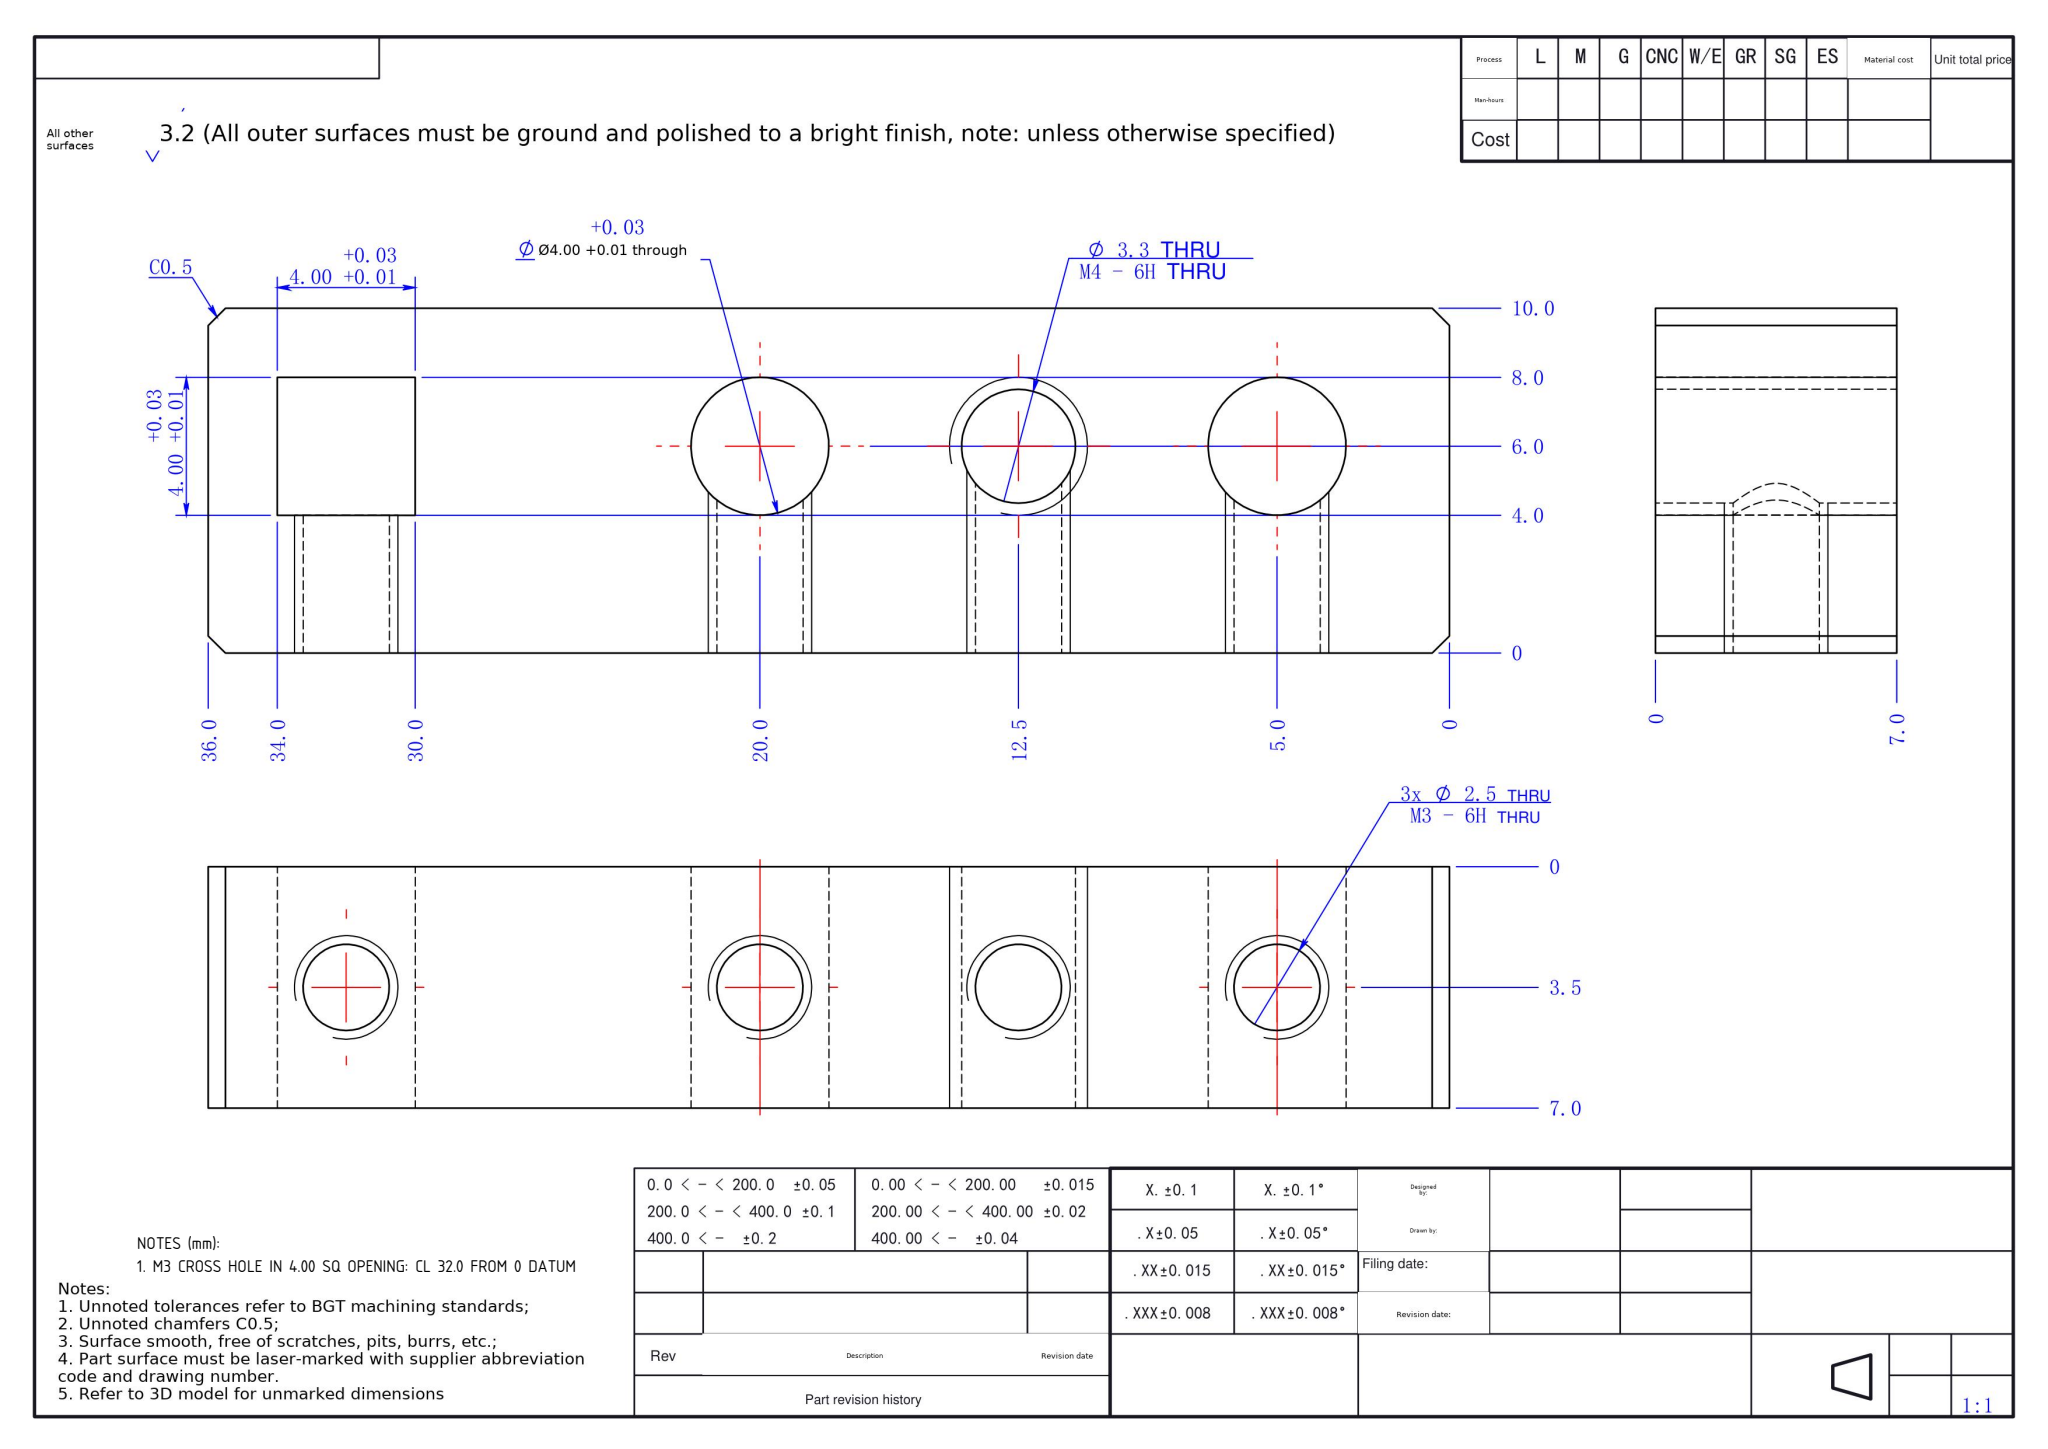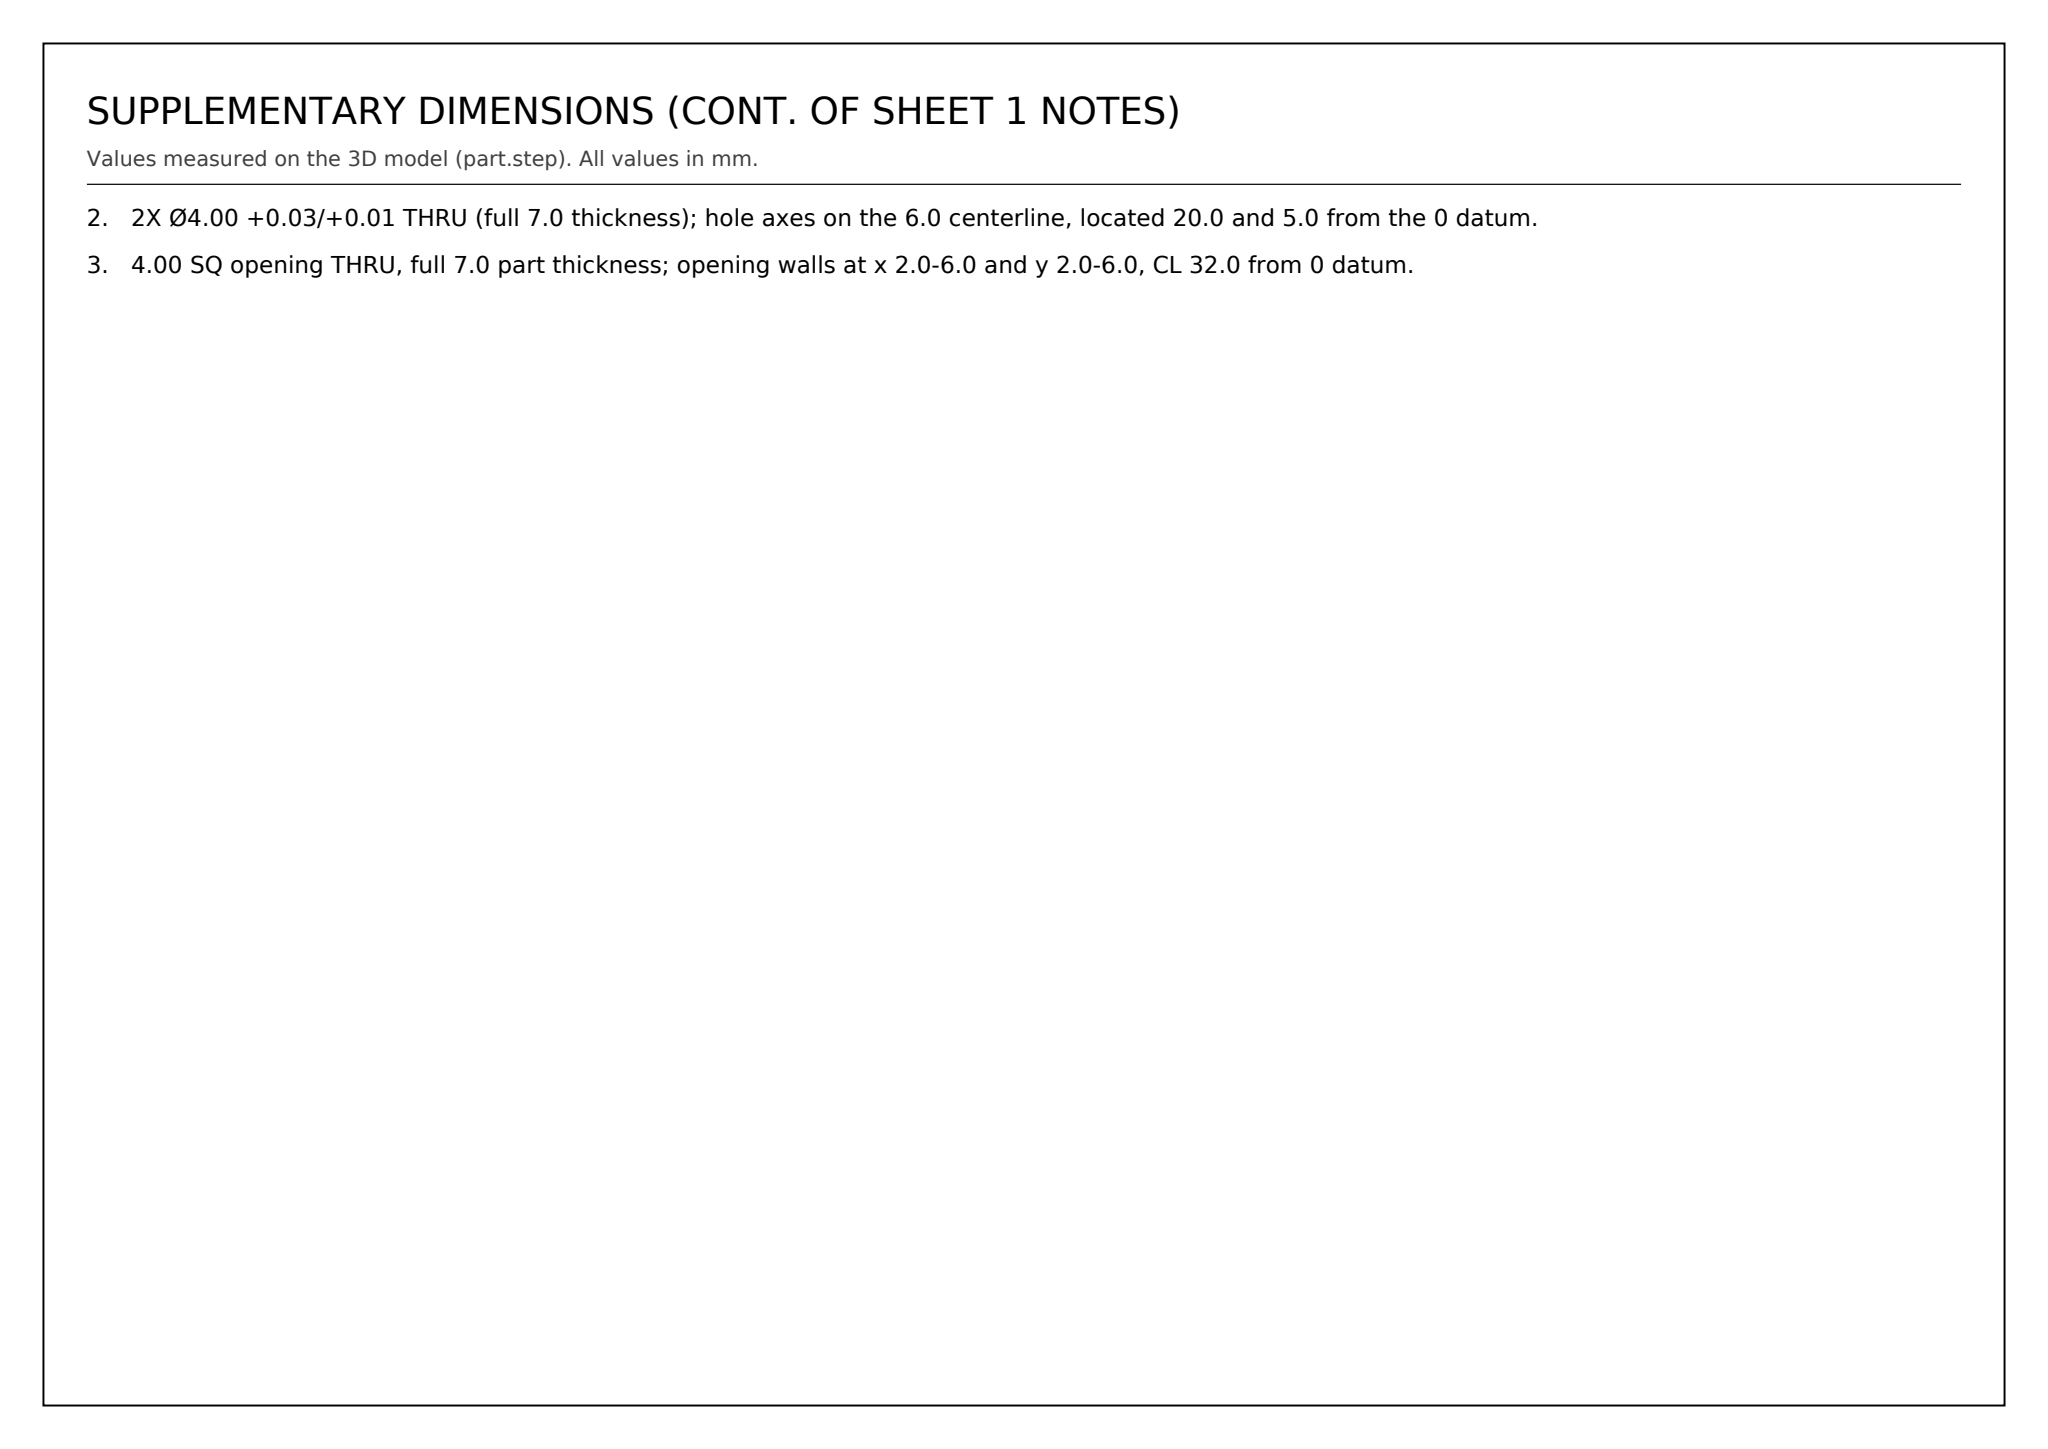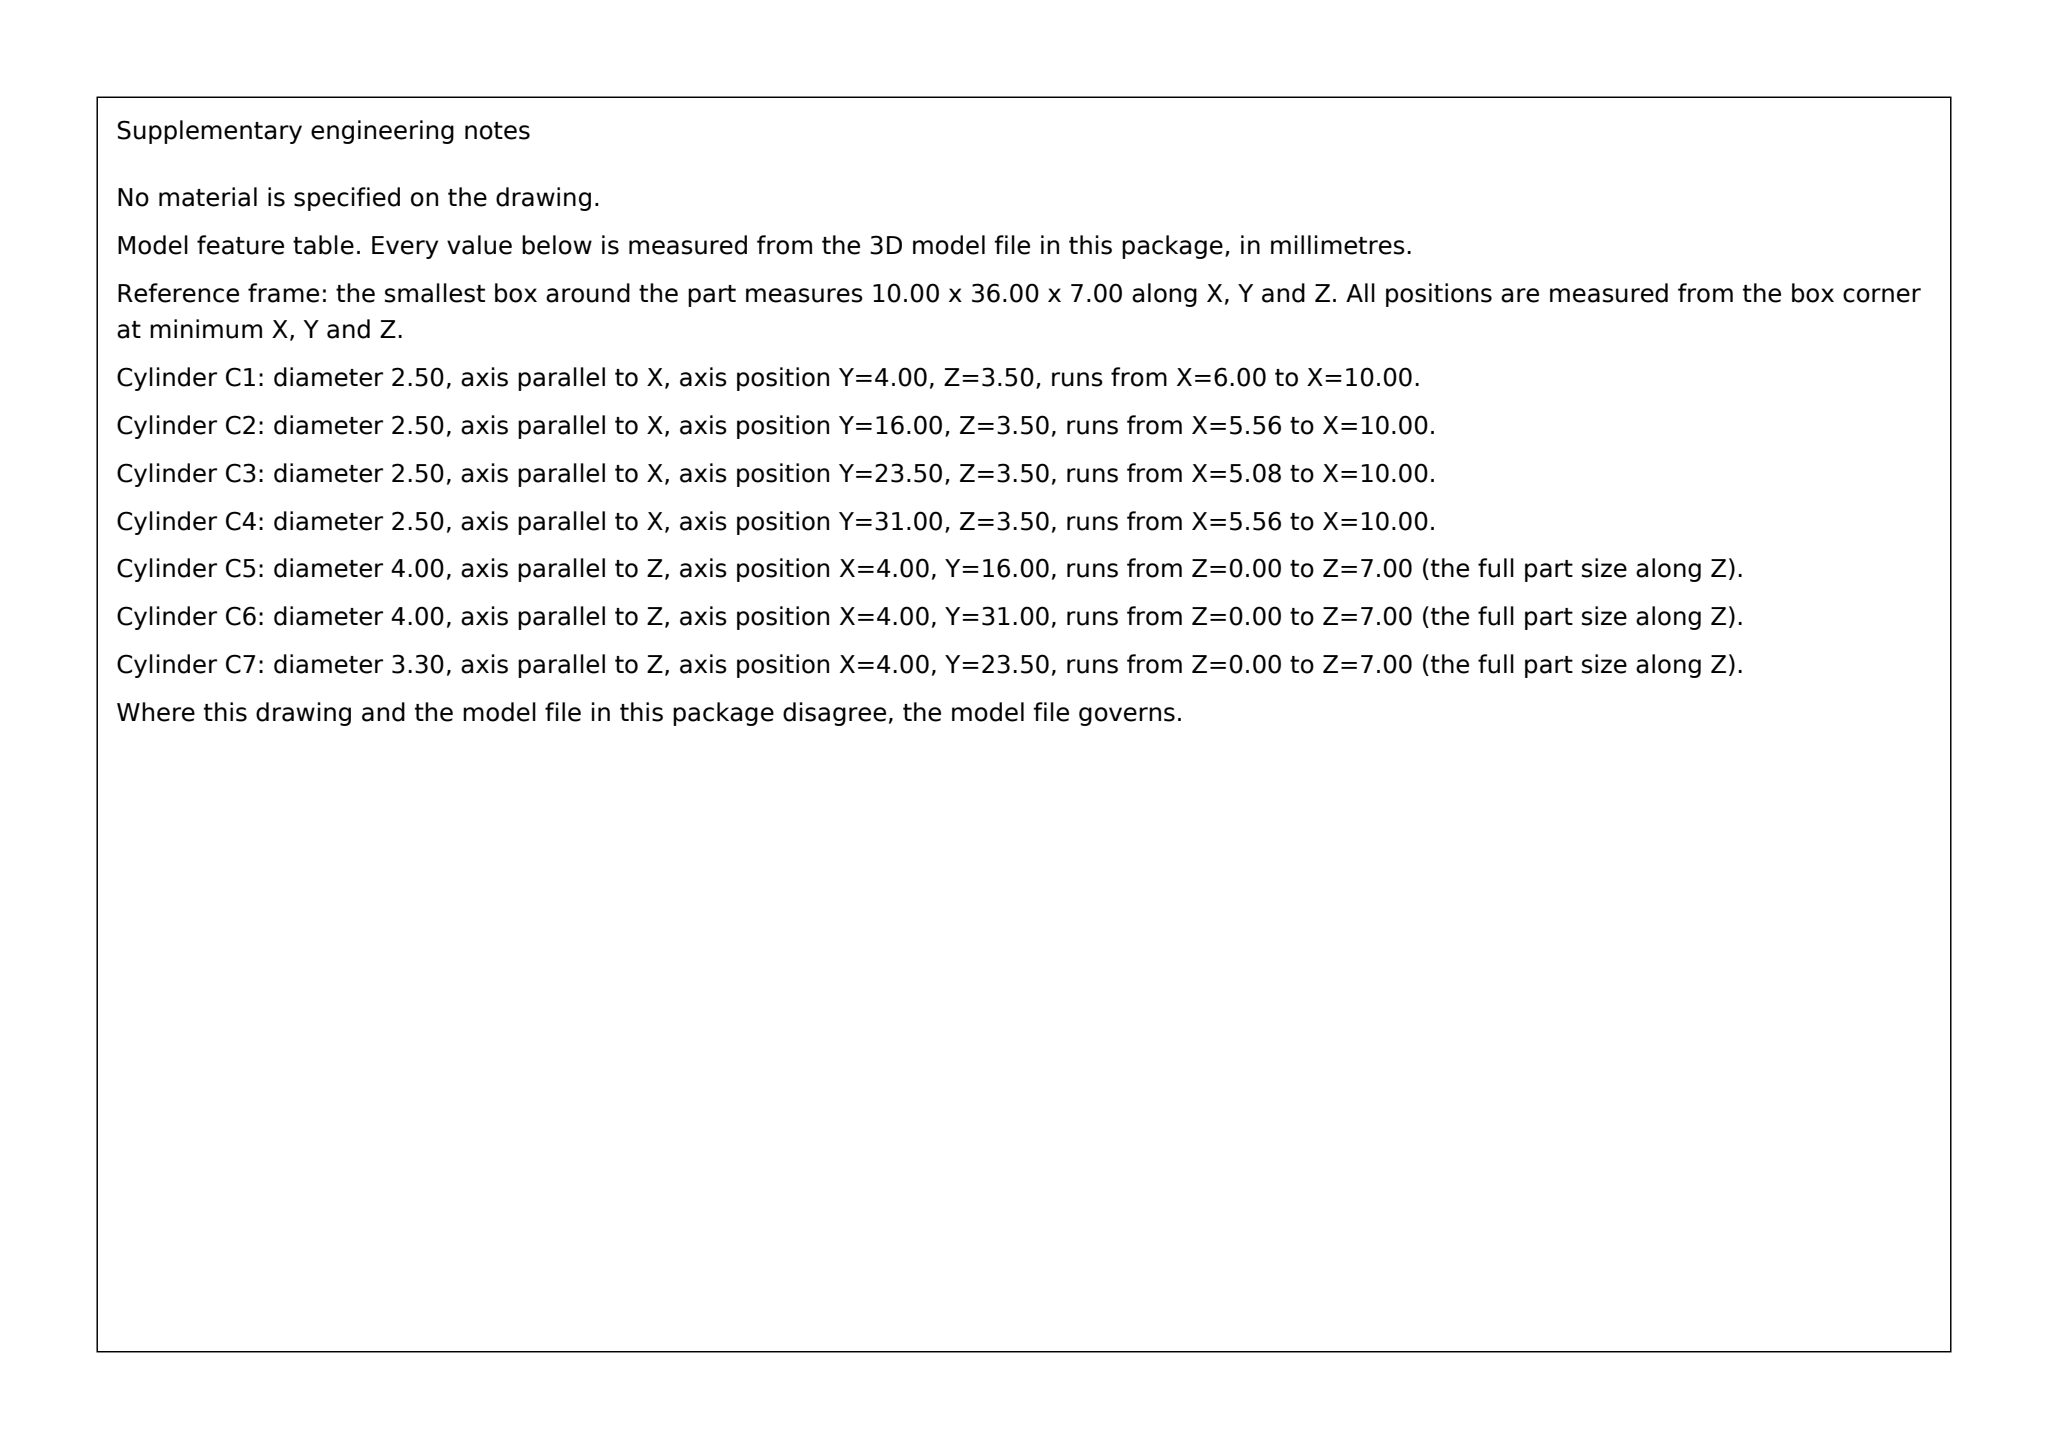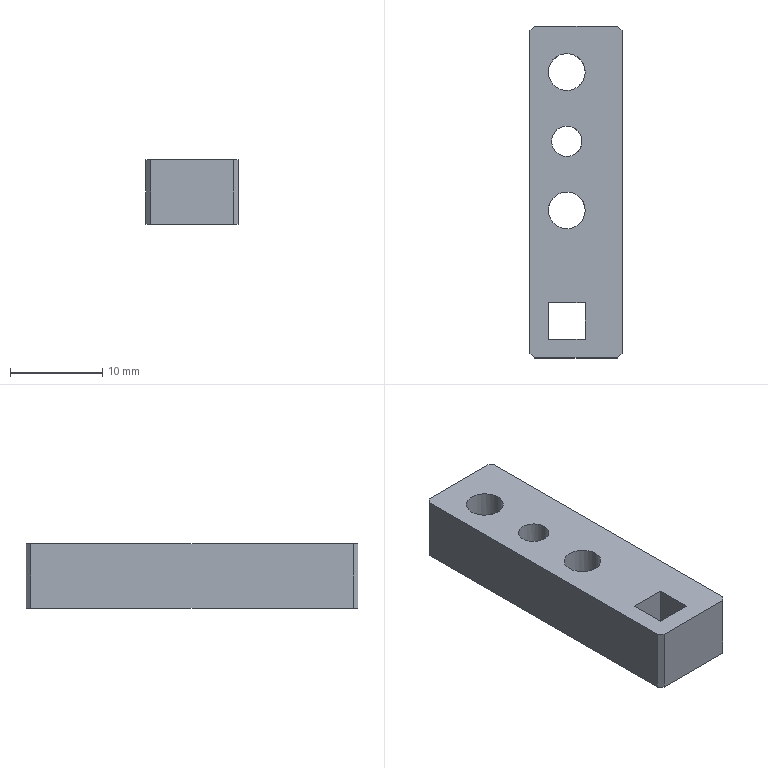Part | SolidWorks | mm | 1 solid | 28 faces | box 10 x 36 x 7 mm | volume 2087 mm3 | cylinder 14 | plane 14 | commonest cylinder face diameters 2.5 x8 4 x4 3.3 x2
Drawing notes:
M3 CROSS HOLE IN 4.00 SQ OPENING: CL 32.0 FROM 0 DATUM | from the solid: dia 2.5 x-axis cylinder at y=4.0, z=3.5; 36.0-4.0=32.0 from right-hand 0 datum, between 30.0 and 34.0
2X Ø4.00 +0.03/+0.01 THRU (full 7.0 thickness); hole axes on the 6.0 centerline, located 20.0 and 5.0 from the 0 datum. | from the solid: cylinders: two 'hole/bore' dia 4.0, axis z, at (x=4.0, y=16.0) and (x=4.0, y=31.0), from z 0.0 to 7.0 (bbox 10.0 x 36.0 x 7.0)
4.00 SQ opening THRU, full 7.0 part thickness; opening walls at x 2.0-6.0 and y 2.0-6.0, CL 32.0 from 0 datum. | from the solid: axis_planes: x=2.0 and x=6.0 and y=2.0 and y=6.0, each with z extent [0.0, 7.0] (square pocket walls spanning full thickness)
build123d program:
from build123d import *

# Parameters (mm, degrees)
SKETCH1_W              = 10
SKETCH1_H              = 36
BOSS_EXTRUDE1_DEPTH    = 7
SKETCH2_W              = 4
SKETCH2_H              = 4
CUT_EXTRUDE1_DEPTH     = 42.838
SKETCH3_R              = 2
CUT_EXTRUDE2_DEPTH     = 42.838
SKETCH4_R              = 1.5
CUT_EXTRUDE3_DEPTH     = 42.838
M3_TAPPED_HOLE1_D      = 2.5
M3_TAPPED_HOLE1_DEPTH  = 4
M3_TAPPED_HOLE1_TIP    = 0.7511
CHAMFER1_SIZE          = 0.5
M3_TAPPED_HOLE2_REACH  = 27.159
M3_TAPPED_HOLE2_BORE_R = 1.25
CHAMFER3_SIZE          = 0.5
M4_TAPPED_HOLE1_D      = 3.3


with BuildPart() as part:
    # Sketch1 → Boss-Extrude1 (new body)
    with BuildSketch(Plane.XY):
        with Locations((-29.892, 4)):
            Rectangle(SKETCH1_W, SKETCH1_H)
    extrude(amount=BOSS_EXTRUDE1_DEPTH)

    # Sketch2 → Cut-Extrude1 (cut, through all)
    with BuildSketch(Plane(origin=(0, 0, 0), x_dir=(-1, 0, 0), z_dir=(0, 0, -1))):
        with Locations((30.892, -10)):
            Rectangle(SKETCH2_W, SKETCH2_H)
    extrude(amount=-CUT_EXTRUDE1_DEPTH, mode=Mode.SUBTRACT)

    # Sketch3 → Cut-Extrude2 (cut, through all)
    with BuildSketch(Plane(origin=(0, 0, 0), x_dir=(-1, 0, 0), z_dir=(0, 0, -1))):
        with Locations((30.892, 2)):
            Circle(SKETCH3_R)
        with Locations((30.892, 17)):
            Circle(SKETCH3_R)
    extrude(amount=-CUT_EXTRUDE2_DEPTH, mode=Mode.SUBTRACT)

    # Sketch4 → Cut-Extrude3 (cut, through all)
    with BuildSketch(Plane(origin=(0, 0, 0), x_dir=(-1, 0, 0), z_dir=(0, 0, -1))):
        with Locations((30.892, 9.5)):
            Circle(SKETCH4_R)
    extrude(amount=-CUT_EXTRUDE3_DEPTH, mode=Mode.SUBTRACT)

    # M3 Tapped Hole1
    with Locations(Plane(origin=(-24.892, 0, 0), x_dir=(0, 0, -1), z_dir=(1, 0, 0))):
        with Locations((-3.5, -10)):
            Hole(M3_TAPPED_HOLE1_D / 2, depth=M3_TAPPED_HOLE1_DEPTH)
            with Locations((0, 0, -(M3_TAPPED_HOLE1_DEPTH + M3_TAPPED_HOLE1_TIP / 2))):  # 118° drill point
                Cone(0, M3_TAPPED_HOLE1_D / 2, M3_TAPPED_HOLE1_TIP, mode=Mode.SUBTRACT)

    # Chamfer1
    chamfer1_edges = [part.edges().sort_by_distance(p)[0] for p in [
        (-34.892, 22, 3.5),
        (-24.892, 22, 3.5),
    ]]
    chamfer(chamfer1_edges, length=CHAMFER1_SIZE)

    # M3 Tapped Hole2 bore → M3 Tapped Hole2 (cut, up to next)
    with BuildSketch(Plane(origin=(-24.892, 0, 0), x_dir=(0, 0, -1), z_dir=(1, 0, 0)), mode=Mode.PRIVATE) as m3_tapped_hole2_sk1:
        with Locations((-3.5, 17)):
            Circle(M3_TAPPED_HOLE2_BORE_R)
    m3_tapped_hole2_tool1 = extrude(m3_tapped_hole2_sk1.sketch, amount=-M3_TAPPED_HOLE2_REACH, mode=Mode.PRIVATE) & part.part
    # M3 Tapped Hole2 bore → M3 Tapped Hole2 (cut, up to next)
    with BuildSketch(Plane(origin=(-24.892, 0, 0), x_dir=(0, 0, -1), z_dir=(1, 0, 0)), mode=Mode.PRIVATE) as m3_tapped_hole2_sk2:
        with Locations((-3.5, 2)):
            Circle(M3_TAPPED_HOLE2_BORE_R)
    m3_tapped_hole2_tool2 = extrude(m3_tapped_hole2_sk2.sketch, amount=-M3_TAPPED_HOLE2_REACH, mode=Mode.PRIVATE) & part.part
    # M3 Tapped Hole2 bore → M3 Tapped Hole2 (cut, up to next)
    with BuildSketch(Plane(origin=(-24.892, 0, 0), x_dir=(0, 0, -1), z_dir=(1, 0, 0)), mode=Mode.PRIVATE) as m3_tapped_hole2_sk3:
        with Locations((-3.5, 9.5)):
            Circle(M3_TAPPED_HOLE2_BORE_R)
    m3_tapped_hole2_tool3 = extrude(m3_tapped_hole2_sk3.sketch, amount=-M3_TAPPED_HOLE2_REACH, mode=Mode.PRIVATE) & part.part
    add(m3_tapped_hole2_tool1.solids().sort_by_distance((-24.892, 17, 3.5))[0], mode=Mode.SUBTRACT)
    add(m3_tapped_hole2_tool2.solids().sort_by_distance((-24.892, 2, 3.5))[0], mode=Mode.SUBTRACT)
    add(m3_tapped_hole2_tool3.solids().sort_by_distance((-24.892, 9.5, 3.5))[0], mode=Mode.SUBTRACT)

    # Chamfer3
    chamfer3_edges = [part.edges().sort_by_distance(p)[0] for p in [
        (-24.892, -14, 3.5),
        (-34.892, -14, 3.5),
    ]]
    chamfer(chamfer3_edges, length=CHAMFER3_SIZE)

    # M4 Tapped Hole1 (through all)
    with Locations(Plane(origin=(0, 0, 0), x_dir=(-1, 0, 0), z_dir=(0, 0, -1))):
        with Locations((30.892, 9.5)):
            Hole(M4_TAPPED_HOLE1_D / 2)


solid = part.part